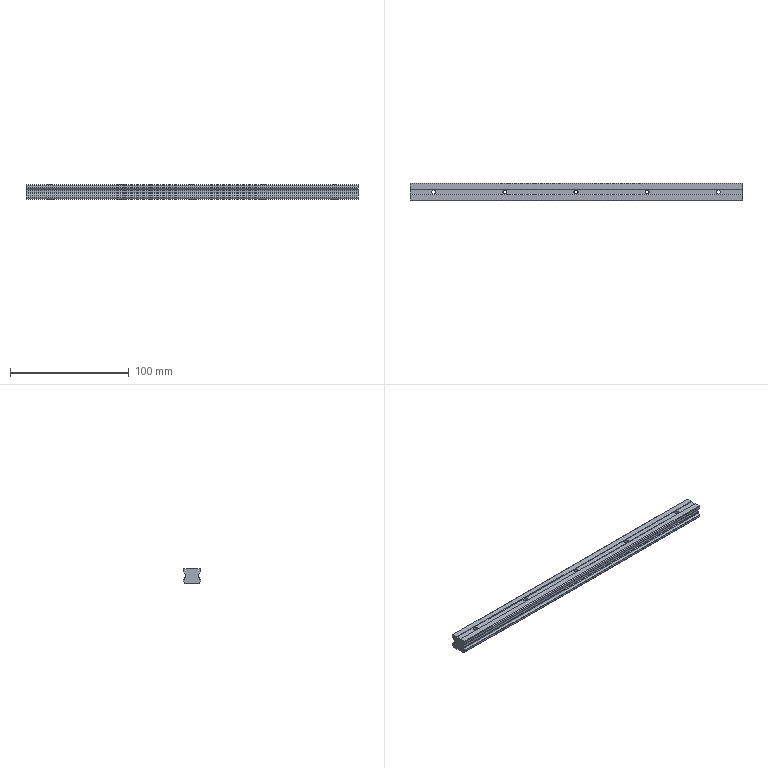Component | SolidWorks | CCDJSBufferChainBlankingLinearGuide-EGH15CA1R160-1_CCDJSBufferChainBlankingLinearGuide-EGR15R160-1 | 1 solid | 62 faces | box 280 x 15 x 12.5 mm | volume 44713 mm3 | cylinder 37 | plane 25 | commonest cylinder face diameters 6 x10 3.5 x10 0.6 x10 3 x5 1 x2 | material AISI 304
build123d program:
from build123d import *

# Parameters (mm, degrees)
BOSS_EXTRUDE1_DEPTH                             = 140
M3_HEX_SOCKET_HEAD_CAP_SCREW_CBORE1_D           = 3.5
M3_HEX_SOCKET_HEAD_CAP_SCREW_CBORE1_CBORE_D     = 6
M3_HEX_SOCKET_HEAD_CAP_SCREW_CBORE1_CBORE_DEPTH = 4.5
LPATTERN1_COUNT                                 = 5
LPATTERN1_PITCH                                 = 60


with BuildPart() as part:
    # Sketch1 → Boss-Extrude1 (new, symmetric)
    with BuildSketch(Plane.XY):
        with BuildLine():
            Line((6.029, 7.336), (5.588, 6.894))
            ThreePointArc((5.588, 6.894), (5.523, 6.797), (5.5, 6.682))
            Line((5.5, 6.682), (5.5, 4.524))
            ThreePointArc((5.5, 4.524), (5.523, 4.409), (5.588, 4.312))
            Line((5.588, 4.312), (7.354, 2.546))
            ThreePointArc((7.354, 2.546), (7.462, 2.384), (7.5, 2.193))
            Line((7.5, 2.193), (7.5, 0.4))
            Line((7.5, 0.4), (6.8, -0.3))
            Line((6.8, -0.3), (2.35, -0.3))
            Line((2.35, -0.3), (2.05, 0))
            Line((2.05, 0), (-2.05, 0))
            Line((-2.05, 0), (-2.35, -0.3))
            Line((-2.35, -0.3), (-6.8, -0.3))
            Line((-6.8, -0.3), (-7.5, 0.4))
            Line((-7.5, 0.4), (-7.5, 2.193))
            ThreePointArc((-7.5, 2.193), (-7.462, 2.384), (-7.354, 2.546))
            Line((-7.354, 2.546), (-5.588, 4.312))
            ThreePointArc((-5.588, 4.312), (-5.523, 4.409), (-5.5, 4.524))
            Line((-5.5, 4.524), (-5.5, 6.682))
            ThreePointArc((-5.5, 6.682), (-5.523, 6.797), (-5.588, 6.894))
            Line((-5.588, 6.894), (-6.029, 7.336))
            ThreePointArc((-6.029, 7.336), (-6.419, 8.38), (-7.422, 8.867))
            ThreePointArc((-7.422, 8.867), (-7.48, 8.961), (-7.5, 9.069))
            Line((-7.5, 9.069), (-7.5, 10.531))
            ThreePointArc((-7.5, 10.531), (-7.48, 10.639), (-7.422, 10.733))
            ThreePointArc((-7.422, 10.733), (-6.468, 11.168), (-6.033, 12.122))
            ThreePointArc((-6.033, 12.122), (-5.939, 12.18), (-5.831, 12.2))
            Line((-5.831, 12.2), (5.831, 12.2))
            ThreePointArc((5.831, 12.2), (5.939, 12.18), (6.033, 12.122))
            ThreePointArc((6.033, 12.122), (6.468, 11.168), (7.422, 10.733))
            ThreePointArc((7.422, 10.733), (7.48, 10.639), (7.5, 10.531))
            Line((7.5, 10.531), (7.5, 9.069))
            ThreePointArc((7.5, 9.069), (7.48, 8.961), (7.422, 8.867))
            ThreePointArc((7.422, 8.867), (6.419, 8.38), (6.029, 7.336))
        make_face()
    extrude(amount=BOSS_EXTRUDE1_DEPTH, both=True)

    # M3 Hex Socket Head Cap Screw CBORE1 (through all)
    with Locations(Plane(origin=(0, 12.2, 0), x_dir=(1, 0, 0), z_dir=(0, 1, 0))):
        with Locations((0, -120)):
            m3_hex_socket_head_cap_screw_cbore1 = CounterBoreHole(M3_HEX_SOCKET_HEAD_CAP_SCREW_CBORE1_D / 2, M3_HEX_SOCKET_HEAD_CAP_SCREW_CBORE1_CBORE_D / 2, M3_HEX_SOCKET_HEAD_CAP_SCREW_CBORE1_CBORE_DEPTH)

    # LPattern1: M3 Hex Socket Head Cap Screw CBORE1 ×5
    with Locations(*[(0, 0, -i * LPATTERN1_PITCH) for i in range(1, LPATTERN1_COUNT)]):
        add(m3_hex_socket_head_cap_screw_cbore1, mode=Mode.SUBTRACT)


solid = part.part

# Placed as in the assembly
solid = solid.moved(Location((-77.1, 426.564, -34.8), (-90, 90, 0)))